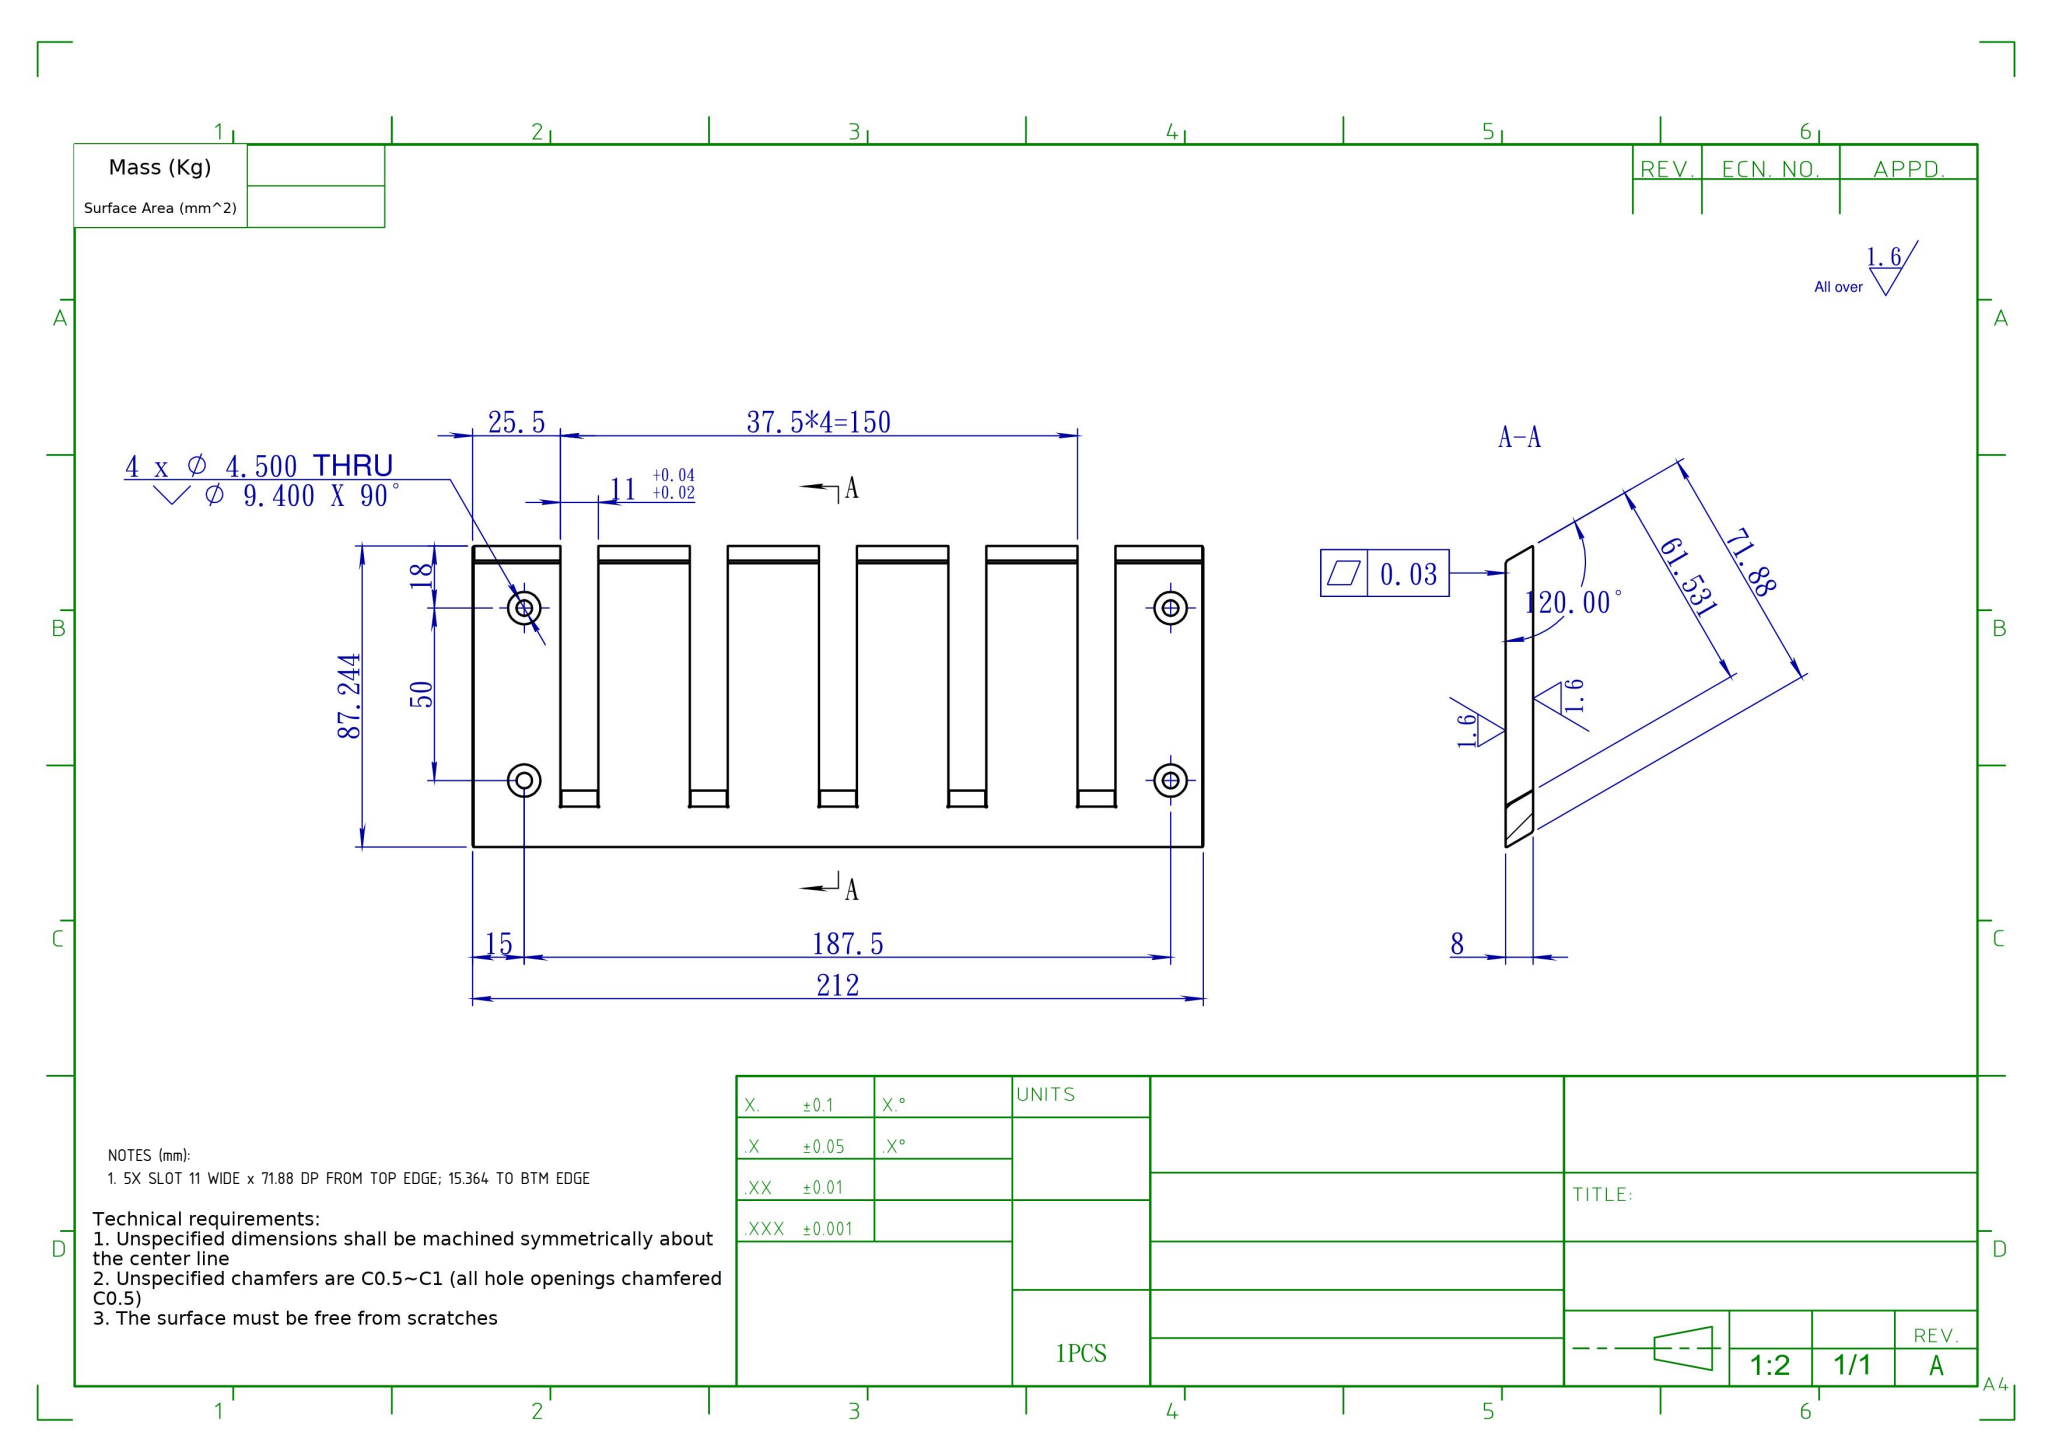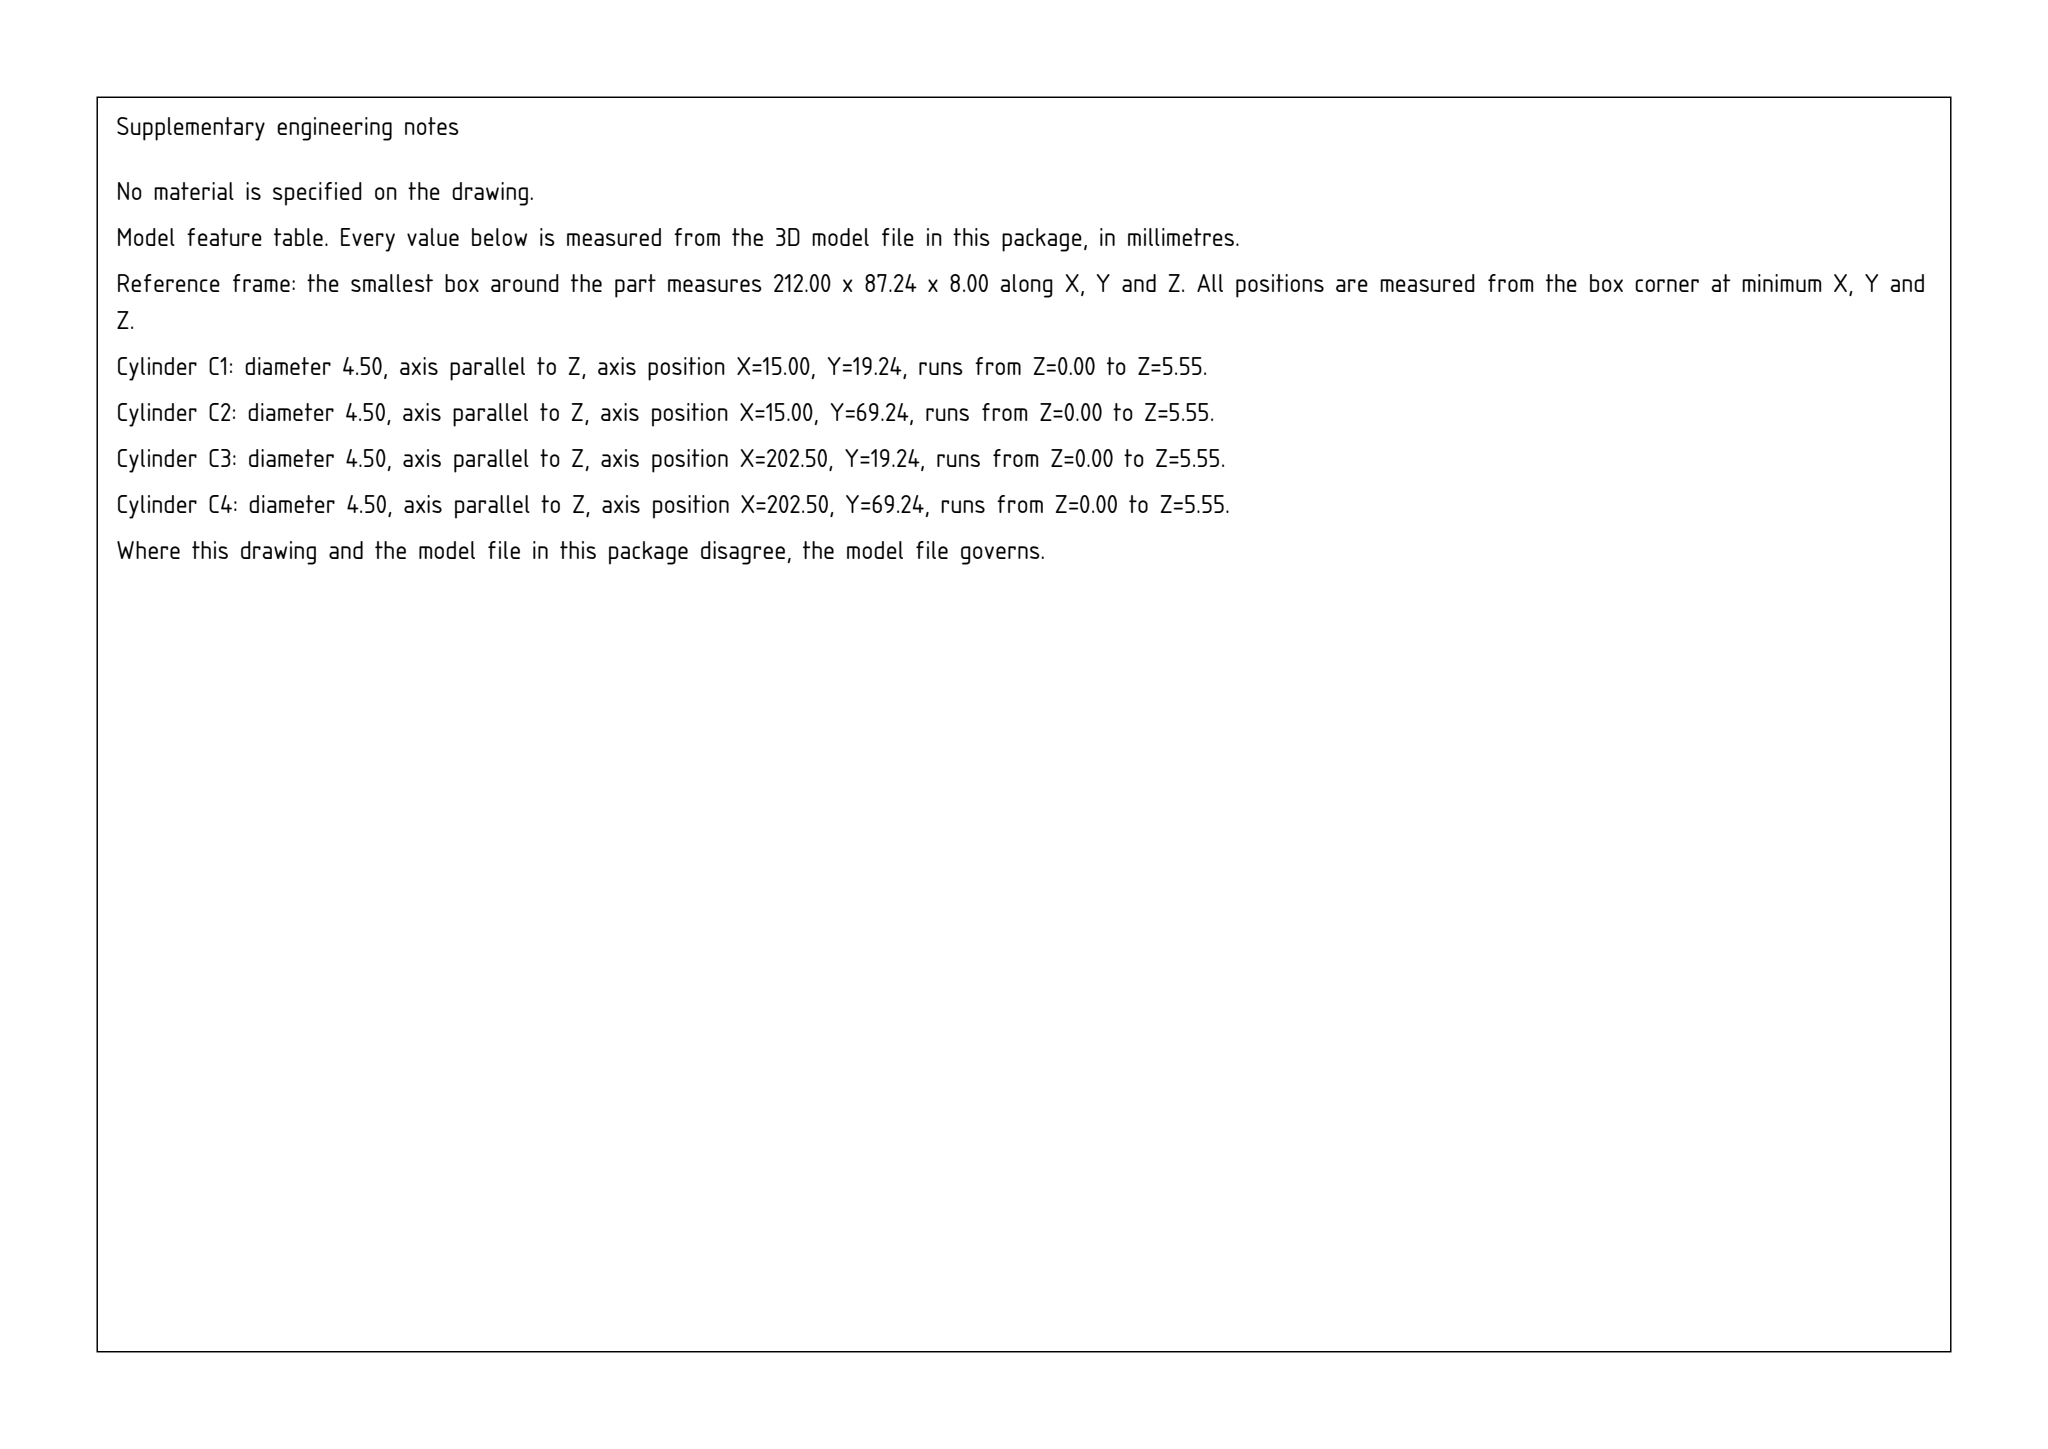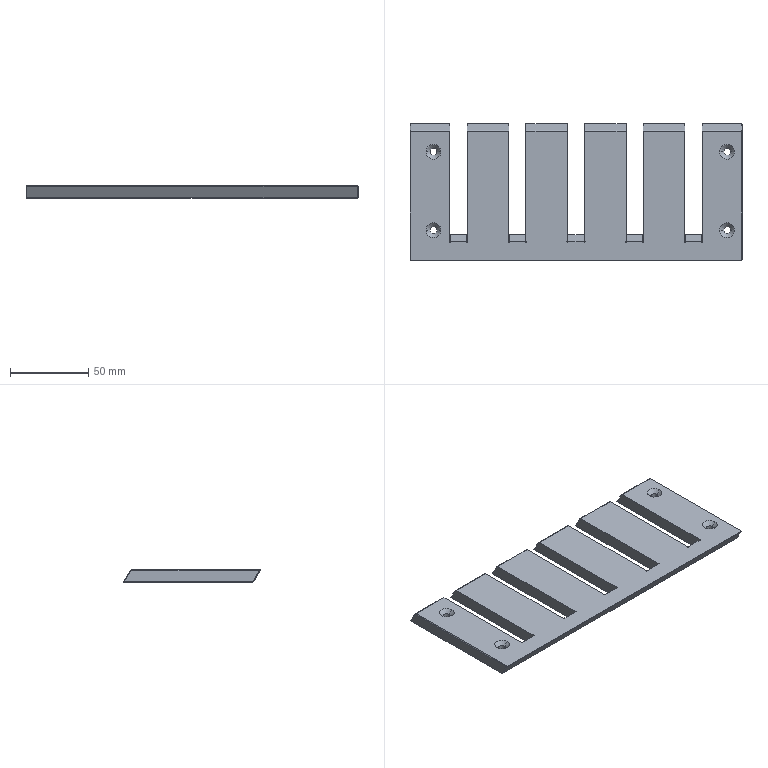Part | SolidWorks | mm | 1 solid | 79 faces | box 212 x 87.24 x 8 mm | volume 108665 mm3 | plane 48 | spline 15 | cone 8 | cylinder 8 | commonest cylinder face diameters 4.5 x8
Drawing notes:
5X SLOT 11 WIDE x 71.88 DP FROM TOP EDGE; 15.364 TO BTM EDGE | from the solid: bbox Y=87.244; slot side planes x 25.5/36.5, 63/74, 100.5/111.5, 138/149, 175.5/186.5 (11 wide, 37.5 pitch); A-A depth 71.88 along slot, leaving 87.244-71.88=15.364 of stock above bottom face y=0
build123d program:
from build123d import *
from OCP.BRepFilletAPI import BRepFilletAPI_MakeChamfer

# Parameters (mm, degrees)
SKETCH1_W                                       = 212
SKETCH1_H                                       = 83
BOSS_EXTRUDE1_DEPTH                             = 8
CUT_EXTRUDE1_DEPTH                              = 217.172
BOSS_EXTRUDE2_DEPTH                             = 212
CHAMFER2_SIZE                                   = 0.5
CHAMFER2_SIZE2                                  = 0.2887
CHAMFER2_SIZE2_2                                = 0.25
CHAMFER3_SIZE                                   = 0.5
CHAMFER3_SIZE2                                  = 0.2887
SKETCH4_W                                       = 11
SKETCH4_H                                       = 78
CUT_EXTRUDE2_DEPTH                              = 116.775
BOSS_EXTRUDE3_DEPTH                             = 11
LINEAR_PATTERN1_COUNT                           = 5
LINEAR_PATTERN1_PITCH                           = 37.5
SKETCH6_R                                       = 0.25
COUNTERSINK_FOR_M4_FLAT_HEAD_SCREW1_D           = 4.5
COUNTERSINK_FOR_M4_FLAT_HEAD_SCREW1_CSINK_D     = 9.4
COUNTERSINK_FOR_M4_FLAT_HEAD_SCREW1_CSINK_ANGLE = 90


with BuildPart() as part:
    # Sketch1 → Boss-Extrude1 (new body)
    with BuildSketch(Plane.XY):
        Rectangle(SKETCH1_W, SKETCH1_H)
    extrude(amount=BOSS_EXTRUDE1_DEPTH)

    # Sketch2 → Cut-Extrude1 (cut, through all)
    with BuildSketch(Plane(origin=(106, 0, 0), x_dir=(0, 0, -1), z_dir=(1, 0, 0))):
        Polygon((0, 41.5), (-8, 36.881), (-8, 41.5), align=None)
    extrude(amount=-CUT_EXTRUDE1_DEPTH, mode=Mode.SUBTRACT)

    # Sketch3 → Boss-Extrude2 (add)
    with BuildSketch(Plane(origin=(106, 0, 0), x_dir=(0, 0, -1), z_dir=(1, 0, 0))):
        Polygon((0, -41.5), (-8, -46.119), (-8, -41.5), align=None)
    extrude(amount=-BOSS_EXTRUDE2_DEPTH)

    # Chamfer2: one chamfer whose edges measure the first distance from different faces: ONE call of the kernel's chamfer builder (chamfer() names one face for all edges)
    chamfer2_edges_1 = [part.edges().sort_by_distance(p)[0] for p in [
        (106, -4.619, 8),
    ]]
    chamfer2_side_1 = [part.faces().sort_by_distance(p)[0] for p in [
        (106, -2.309, 4),
    ]]
    chamfer2_edges_2 = [part.edges().sort_by_distance(p)[0] for p in [
        (-106, -4.619, 8),
    ]]
    chamfer2_side_2 = [part.faces().sort_by_distance(p)[0] for p in [
        (-106, -2.309, 4),
    ]]
    chamfer2_edges_3 = [part.edges().sort_by_distance(p)[0] for p in [
        (0, 36.881, 8),
        (0, -41.5, 0),
    ]]
    chamfer2_edges_4 = [part.edges().sort_by_distance(p)[0] for p in [
        (0, -46.119, 8),
    ]]
    chamfer2_side_4 = [part.faces().sort_by_distance(p)[0] for p in [
        (0, -43.809, 4),
    ]]
    chamfer2_edges_5 = [part.edges().sort_by_distance(p)[0] for p in [
        (0, 41.5, 0),
    ]]
    chamfer2_side_5 = [part.faces().sort_by_distance(p)[0] for p in [
        (0, 0, 0),
    ]]
    chamfer2_edges_6 = [part.edges().sort_by_distance(p)[0] for p in [
        (106, 0, 0),
        (-106, 0, 0),
    ]]
    chamfer2_side_6 = [part.faces().sort_by_distance(p)[0] for p in [
        (0, 0, 0),
    ]]
    chamfer2 = BRepFilletAPI_MakeChamfer(part.part.solid().wrapped)
    for e in chamfer2_edges_1:
        chamfer2.Add(CHAMFER2_SIZE, CHAMFER2_SIZE2, e.wrapped, chamfer2_side_1[0].wrapped)  # the first distance lies on this face
    for e in chamfer2_edges_2:
        chamfer2.Add(CHAMFER2_SIZE, CHAMFER2_SIZE2, e.wrapped, chamfer2_side_2[0].wrapped)  # the first distance lies on this face
    for e in chamfer2_edges_3:
        chamfer2.Add(CHAMFER2_SIZE, e.wrapped)
    for e in chamfer2_edges_4:
        chamfer2.Add(CHAMFER2_SIZE, CHAMFER2_SIZE2_2, e.wrapped, chamfer2_side_4[0].wrapped)  # the first distance lies on this face
    for e in chamfer2_edges_5:
        chamfer2.Add(CHAMFER2_SIZE, CHAMFER2_SIZE2_2, e.wrapped, chamfer2_side_5[0].wrapped)  # the first distance lies on this face
    for e in chamfer2_edges_6:
        chamfer2.Add(CHAMFER2_SIZE, CHAMFER2_SIZE2, e.wrapped, chamfer2_side_6[0].wrapped)  # the first distance lies on this face
    add(Compound.cast(chamfer2.Shape()), mode=Mode.REPLACE)

    # Chamfer3: one chamfer whose edges measure the first distance from different faces: ONE call of the kernel's chamfer builder (chamfer() names one face for all edges)
    chamfer3_edges_1 = [part.edges().sort_by_distance(p)[0] for p in [
        (106, -43.79, 3.967),
    ]]
    chamfer3_side_1 = [part.faces().sort_by_distance(p)[0] for p in [
        (0, -43.809, 4),
    ]]
    chamfer3_edges_2 = [part.edges().sort_by_distance(p)[0] for p in [
        (106, 39.252, 3.894),
    ]]
    chamfer3_side_2 = [part.faces().sort_by_distance(p)[0] for p in [
        (106, -2.248, 3.894),
    ]]
    chamfer3_edges_3 = [part.edges().sort_by_distance(p)[0] for p in [
        (-106, -43.79, 3.967),
    ]]
    chamfer3_side_3 = [part.faces().sort_by_distance(p)[0] for p in [
        (-106, -2.248, 3.894),
    ]]
    chamfer3_edges_4 = [part.edges().sort_by_distance(p)[0] for p in [
        (-106, 39.252, 3.894),
    ]]
    chamfer3_side_4 = [part.faces().sort_by_distance(p)[0] for p in [
        (0, 39.253, 3.892),
    ]]
    chamfer3 = BRepFilletAPI_MakeChamfer(part.part.solid().wrapped)
    for e in chamfer3_edges_1:
        chamfer3.Add(CHAMFER3_SIZE, CHAMFER3_SIZE2, e.wrapped, chamfer3_side_1[0].wrapped)  # the first distance lies on this face
    for e in chamfer3_edges_2:
        chamfer3.Add(CHAMFER3_SIZE, CHAMFER3_SIZE2, e.wrapped, chamfer3_side_2[0].wrapped)  # the first distance lies on this face
    for e in chamfer3_edges_3:
        chamfer3.Add(CHAMFER3_SIZE, CHAMFER3_SIZE2, e.wrapped, chamfer3_side_3[0].wrapped)  # the first distance lies on this face
    for e in chamfer3_edges_4:
        chamfer3.Add(CHAMFER3_SIZE, CHAMFER3_SIZE2, e.wrapped, chamfer3_side_4[0].wrapped)  # the first distance lies on this face
    add(Compound.cast(chamfer3.Shape()), mode=Mode.REPLACE)

    # Sketch4 → Cut-Extrude2 (cut, through all)
    with BuildSketch(Plane.XY.offset(8)):
        with Locations((75, 3.131)):
            Rectangle(SKETCH4_W, SKETCH4_H)
        with Locations((37.5, 3.131)):
            Rectangle(SKETCH4_W, SKETCH4_H)
        with Locations((0, 3.131)):
            Rectangle(SKETCH4_W, SKETCH4_H)
        with Locations((-37.5, 3.131)):
            Rectangle(SKETCH4_W, SKETCH4_H)
        with Locations((-75, 3.131)):
            Rectangle(SKETCH4_W, SKETCH4_H)
    extrude(amount=-CUT_EXTRUDE2_DEPTH, mode=Mode.SUBTRACT)

    # Sketch5 → Boss-Extrude3 (add)
    with BuildSketch(Plane(origin=(69.5, 0, 0), x_dir=(0, 0, -1), z_dir=(1, 0, 0))):
        Polygon((-8, -35.869), (0, -35.869), (0, -29.55), (-8, -34.169), align=None)
    boss_extrude3 = extrude(amount=BOSS_EXTRUDE3_DEPTH)

    # Linear Pattern1: Boss-Extrude3 ×5
    with Locations(*[(-i * LINEAR_PATTERN1_PITCH, 0, 0) for i in range(1, LINEAR_PATTERN1_COUNT)]):
        add(boss_extrude3)

    # Cut-Sweep1: sweep along a curve in space
    with BuildLine() as cut_sweep1_path:
        Line((69.5, -29.55, 0), (69.5, -34.169, 8))
    # Sketch6 → Cut-Sweep1 (sweep, cut)
    with BuildSketch(Plane.XY.offset(8)):
        with Locations((80.5, -34.169)):
            Circle(SKETCH6_R)
        with Locations((69.5, -34.169)):
            Circle(SKETCH6_R)
        with Locations((43, -34.169)):
            Circle(SKETCH6_R)
        with Locations((32, -34.169)):
            Circle(SKETCH6_R)
        with Locations((5.5, -34.169)):
            Circle(SKETCH6_R)
        with Locations((-5.5, -34.169)):
            Circle(SKETCH6_R)
        with Locations((-32, -34.169)):
            Circle(SKETCH6_R)
        with Locations((-43, -34.169)):
            Circle(SKETCH6_R)
        with Locations((-69.5, -34.169)):
            Circle(SKETCH6_R)
        with Locations((-80.5, -34.169)):
            Circle(SKETCH6_R)
    sweep(path=cut_sweep1_path.line, mode=Mode.SUBTRACT)

    # Countersink for M4 Flat Head Screw1 (through all)
    with Locations(Plane.XY.offset(8)):
        with Locations((-91, 23.375), (-91, -26.625), (96.5, 23.375), (96.5, -26.625)):
            CounterSinkHole(COUNTERSINK_FOR_M4_FLAT_HEAD_SCREW1_D / 2, COUNTERSINK_FOR_M4_FLAT_HEAD_SCREW1_CSINK_D / 2, counter_sink_angle=COUNTERSINK_FOR_M4_FLAT_HEAD_SCREW1_CSINK_ANGLE)


solid = part.part